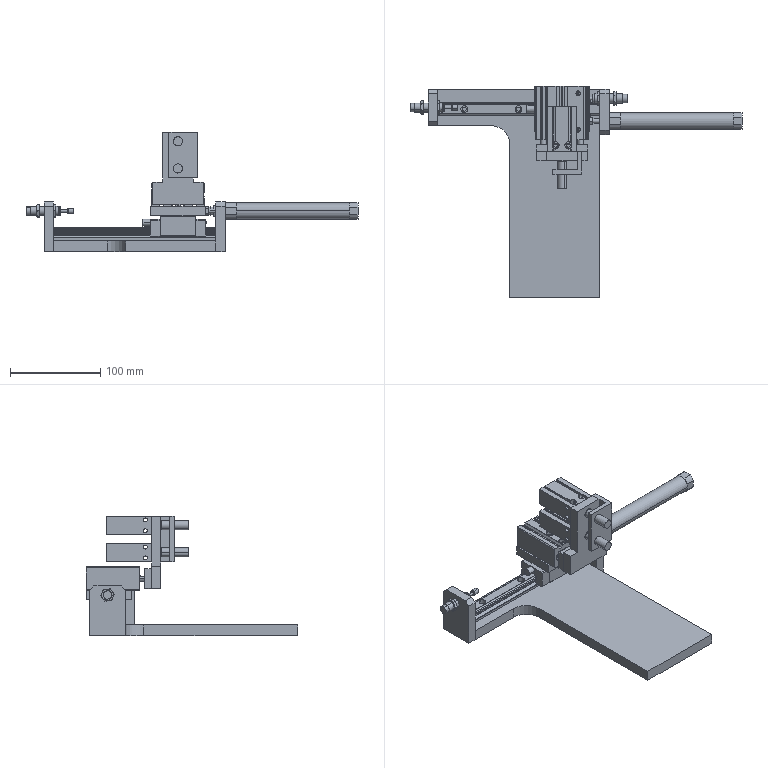Assembly | SolidWorks | mm | 19 component files | 21 solids | 1550 faces | box 367 x 233.3 x 132 mm | volume 687228 mm3 | plane 749 | cylinder 472 | cone 204 | spline 107 | torus 18 | commonest cylinder face diameters 7.6 x40 4.5 x38 10 x36 0.8 x36 5 x30 3 x29 6 x26 4 x24
Bill of materials:
01 | 1 |  | Flat L-shaped plate of uniform thickness with a single rounded (filleted) inside corner.
02 | 1 |  | Rectangular block/thick plate with two round holes entering one long side face.
03 | 1 |  | Flat T-shaped plate made of a wide rectangular base with a narrower upright tab; the tab has two through holes in a line.
04 | 1 |  | Angle bracket with two legs at a right angle; one leg has two through holes.
05 | 2 |  | Plain solid cylinder (round rod or pin) with flat ends.
06 | 1 |  | Rectangular plate with both top corners chamfered and a single round through hole centered near the chamfered edge.
07 | 1 |  | Rectangular plate with both top corners chamfered and two round through holes side by side near the chamfered edge.
Buffer | 2 |  | Slender stepped cylindrical body with two hexagonal nuts on the main barrel. A short, smaller-diameter shoulder at one end leads to a thin rod that ends in a short, larger-diameter cylindrical tip. The opposite end has a short, smaller-diameter cylindrical step.
CDJ2B16-100-C73L Retracted | 1 |  | Long, slender cylindrical tube body. Both ends have short collars with flats, about the same diameter as the tube; one collar looks cylindrical in the axial view. A stepped smaller boss at one end carries a thin rod with a small hex nut and a short cylindrical tip.
CDU16-10D-A93L Retract | 2 |  | Compact rectangular block with two long grooves along its top face. It has several round holes, including counterbored holes at the corners that break through the grooves and edges. A stepped cylindrical rod with a hex nut comes out of one end face.
LinearGuideHIWINHG15R150-C | 1 |  | Long straight profiled rail with a constant cross-section that has a groove along each side, and a row of evenly spaced vertical counterbored holes along the top.
SliderHIWINHGH15CA-C | 1 |  | Rectangular block with a downward-facing channel shaped to match a grooved rail, end caps, four threaded-looking or plain holes on the top face, and a small cylindrical stub sticking out of one end.
TC_L_12x30_30fp | 1 |  | Rectangular plate with two parallel round rods sticking out at right angles from one face; the plate carries several holes and socket-head features.
TC_L_12x30_30r | 1 |  | Stepped cylindrical pin or shaft with a long slender shank, a small reduced-diameter tip with an axial bore, and a head made of several stacked collars/flanges with grooves between them.
TC_L_12x3030_b | 1 |  | Block cut from a multi-slot extruded profile, with T-slots and V-grooves on its outer faces, through bores along its length, counterbored holes through the top, and plugs with hex sockets on a side face.
TCL_TCM_12_Screw | 1 |  | Socket-head-cap-screw-like solid: a short cylindrical head with a hexagonal socket recess in its end face, joined to a longer plain cylindrical shank that ends in a chamfer. No threads are modeled.
Mates:
1. coincident | CDUSeriesCylinder-1 face at (-58, 211.3, 86) dir (-1, 0, 0) | CDUSeriesCylinder-2 face at (-58, 211.3, 116) dir (-1, 0, 0)
2. concentric | 04-1 face at (-42, 136.3, 116) dir (0, 1, 0) r 5 | 05-1 face at (-42, 150.3, 116) dir (0, -1, 0) r 5
3. coincident | CDUSeriesCylinder-2 face at (-42, 150.3, 116) dir (0, -1, 0) | 05-1 face at (-42, 150.3, 116) dir (0, 1, 0)
4. coincident | CDUSeriesCylinder-1 face at (-42, 150.3, 86) dir (0, -1, 0) | 05-2 face at (-42, 150.3, 86) dir (0, 1, 0)
5. concentric | 04-1 face at (-42, 136.3, 86) dir (0, 1, 0) r 5 | 05-2 face at (-42, 150.3, 86) dir (0, -1, 0) r 5
6. concentric | 07-1 face at (10, 195, 39) dir (-1, 0, 0) r 5 | CDJ2BSeries-1 face at (-18, 195, 39) dir (1, 0, 0) r 9.15
7. coincident | 07-1 face at (10, 0, 0) dir (1, 0, 0) | CDJ2BSeries-1 face at (10, 200, 39) dir (-1, 0, 0)
8. concentric | 06-1 face at (-190, 210, 39) dir (1, 0, 0) r 5 | Buffer-1 face at (-157, 210, 39) dir (1, 0, 0) r 5
9. concentric | 07-1 face at (10, 220, 39) dir (-1, 0, 0) r 5 | Buffer-2 face at (-23, 220, 39) dir (-1, 0, 0) r 5
10. coincident | 07-1 face at (0, 0, 0) dir (-1, 0, 0) | Buffer-2 face at (0, 225, 39) dir (1, 0, 0)
11. coincident | SliderHIWINHGH15CA-C-1 face at (-61.7, 203.251, 21) dir (0, 0, -1) | LinearGuideHIWINHG15R150-C-1 face at (-165, 213.349, 21) dir (0, 0, 1)
12. coincident | SliderHIWINHGH15CA-C-1 face at (-61.7, 215.8, 18.549) dir (0, -1, 0) | LinearGuideHIWINHG15R150-C-1 face at (-165, 215.8, 17.011) dir (0, 1, 0)
13. coincident | 01-1 face at (0, 0, 6) dir (0, 0, 1) | LinearGuideHIWINHG15R150-C-1 face at (-165, 201.5, 6) dir (0, 0, -1)
14. distance | SliderHIWINHGH15CA-C-1 face at (-61.7, 225, 11.3) dir (0, 1, 0) | 01-1 face at (0, 230, 6) dir (0, 1, 0)
15. coincident | 01-1 face at (0, 0, 6) dir (1, 0, 0) | LinearGuideHIWINHG15R150-C-1 face at (0, 208.3, 21) dir (1, 0, 0)
16. coincident | 02-1 face at (-42, 208.3, 34) dir (0, 0, -1) | SliderHIWINHGH15CA-C-1 face at (-61.7, 199.3, 34) dir (0, 0, 1)
17. coincident | 02-1 plane at (-42, 208.3, 39) dir (-1, 0, 0) | SliderHIWINHGH15CA-C-1 plane at (-42, 208.3, 21) dir (1, 0, 0)
18. coincident | 02-1 plane at (-42, 208.3, 39) dir (0, 1, 0) | SliderHIWINHGH15CA-C-1 plane at (-42, 208.3, 21) dir (0, 1, 0)
19. coincident | 02-1 face at (-42, 208.3, 44) dir (0, 0, 1) | TC_L_12x30_S_0-1/TC_L_12x3030_b-1 face at (-49, 233.3, 44) dir (0, 0, -1)
20. coincident | 02-1 face at (-12, 233.3, 34) dir (0, 1, 0) | TC_L_12x30_S_0-1/TC_L_12x3030_b-1 face at (-21.1, 233.3, 45.8) dir (0, 1, 0)
21. coincident | 02-1 plane at (-42, 208.3, 39) dir (-1, 0, 0) | TC_L_12x30_S_0-1 plane at (-42, 174.3, 57) dir (-1, 0, 0)
22. coincident | 03-1 face at (-42, 161.3, 86) dir (0, 1, 0) | TC_L_12x30_S_0-1/TC_L_12x30_30fp-1 face at (-42, 161.3, 57) dir (0, -1, 0)
23. coincident | 03-1 face at (-70, 161.3, 46) dir (0, 0, -1) | TC_L_12x30_S_0-1/TC_L_12x30_30fp-1 face at (-14.2, 169.3, 46) dir (0, 0, -1)
24. coincident | 02-1 plane at (-42, 208.3, 39) dir (-1, 0, 0) | 03-1 plane at (-42, 156.3, 86) dir (1, 0, 0)
25. coincident | 03-1 face at (-42, 161.3, 86) dir (0, 1, 0) | CDUSeriesCylinder-2 face at (-42, 161.3, 116) dir (0, -1, 0)
26. coincident | 03-1 face at (-42, 161.3, 86) dir (0, 1, 0) | CDUSeriesCylinder-1 face at (-42, 161.3, 86) dir (0, -1, 0)
27. concentric | 03-1 face at (-42, 161.3, 116) dir (0, -1, 0) r 5 | CDUSeriesCylinder-2 face at (-42, 186.3, 116) dir (0, 1, 0) r 2.5
28. concentric | CDUSeriesCylinder-2 face at (-42, 186.3, 116) dir (0, 1, 0) r 2.5 | 05-1 face at (-42, 150.3, 116) dir (0, -1, 0) r 5
29. concentric | CDUSeriesCylinder-1 face at (-42, 186.3, 86) dir (0, 1, 0) r 2.5 | 05-2 face at (-42, 150.3, 86) dir (0, -1, 0) r 5
30. coincident | 03-1 face at (-70, 161.3, 126) dir (0, 0, 1) | CDUSeriesCylinder-2 face at (-42, 211.3, 126) dir (0, 0, 1)
31. coincident | 02-1 face at (-12, 183.3, 34) dir (1, 0, 0) | CDJ2BSeries-1 face at (-12, 199, 39) dir (-1, 0, 0)
32. coincident | 06-1 face at (-180, 0, 6) dir (1, 0, 0) | Buffer-1 face at (-180, 208.091, 43.621) dir (-1, 0, 0)
33. coincident | 03-1 face at (-42, 161.3, 86) dir (0, 1, 0) | 04-1 face at (-20, 161.3, 126) dir (0, 1, 0)
34. coincident | TC_L_12x3030_b-1 axis at (-80.9, 0, 0) dir (1, 0, 0) | TC_L_12x30_30fp-1 axis at (67.9, 0, 0) dir (-1, 0, 0)
35. coincident | TC_L_12x3030_b-1 axis at (-80.9, 0, 0) dir (1, 0, 0) | TC_L_12x30_30fp-1 axis at (67.9, 0, 0) dir (-1, 0, 0)
36. coincident | TC_L_12x3030_b-1 axis at (-80.9, 0, 0) dir (1, 0, 0) | TC_L_12x30_30fp-1 axis at (67.9, 0, 0) dir (-1, 0, 0)
37. angle | TC_L_12x30_30fp-1 plane at (-13, 0, 0) dir (0, 1, 0) | TC_L_12x3030_b-1 plane at (0, 0, 0) dir (0, 1, 0)
38. distance | TC_L_12x30_30r-1 plane at (-5, 0, 0) dir (1, 0, 0) | TC_L_12x30_30fp-1 plane at (-5, 0, 0) dir (-1, 0, 0)
39. coincident | TC_L_12x30_30fp-1 axis at (-93.9, 0, 0) dir (1, 0, 0) | TC_L_12x30_30r-1 axis at (75.9, 0, 0) dir (-1, 0, 0)
40. coincident | TC_L_12x30_30fp-1 axis at (-93.9, 0, 0) dir (1, 0, 0) | TC_L_12x30_30r-1 axis at (75.9, 0, 0) dir (-1, 0, 0)
41. angle | TC_L_12x30_30r-1 plane at (-5, 0, 0) dir (0, 0, -1) | TC_L_12x30_30fp-1 plane at (-13, 0, 0) dir (0, 1, 0)
42. distance | TCL_TCM_12_Screw-1 plane at (-10, 0, 0) dir (1, 0, 0) | TC_L_12x30_30fp-1 plane at (-10, 0, 0) dir (-1, 0, 0)
43. coincident | TC_L_12x30_30fp-1 axis at (-93.9, 0, 0) dir (1, 0, 0) | TCL_TCM_12_Screw-1 axis at (70.9, 0, 0) dir (-1, 0, 0)
44. coincident | TC_L_12x30_30fp-1 axis at (-93.9, 0, 0) dir (1, 0, 0) | TCL_TCM_12_Screw-1 axis at (70.9, 0, 0) dir (-1, 0, 0)
45. coincident | TC_L_12x30_30fp-1 axis at (-93.9, 0, 0) dir (1, 0, 0) | TCL_TCM_12_Screw-1 axis at (70.9, 0, 0) dir (-1, 0, 0)
46. angle | TCL_TCM_12_Screw-1 plane at (-10, 0, 0) dir (0, 1, 0) | TC_L_12x30_30fp-1 plane at (-13, 0, 0) dir (0, 1, 0)
47. distance | TC_L_12x30_30fp-1 face at (-5, 0, 0) dir (1, 0, 0) | TC_L_12x3030_b-1 face at (0, -20.9, -11.2) dir (-1, 0, 0)